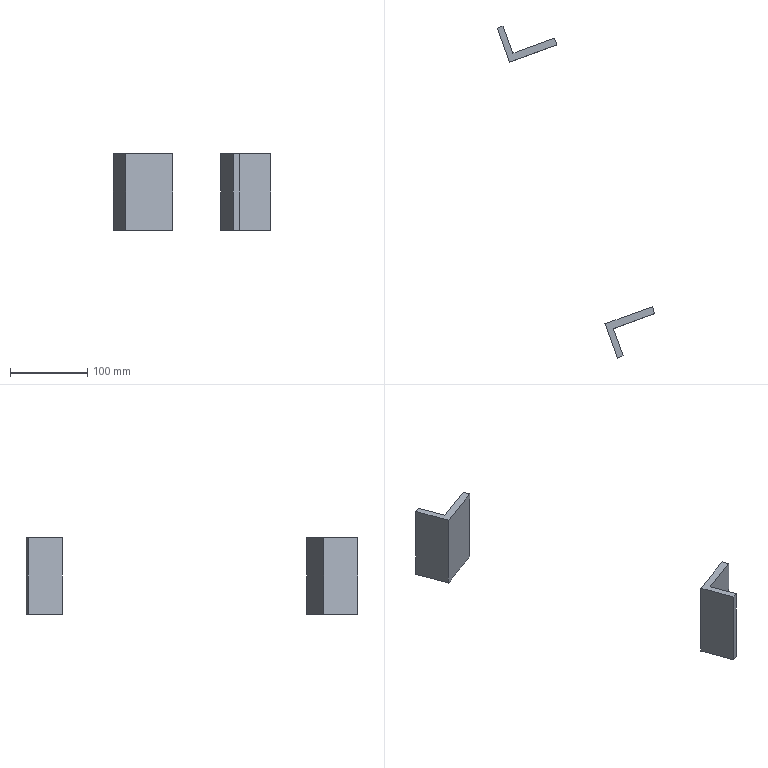Component | NX | MOUNTING_PLATE_2 | 2 solids | 16 faces | box 203.45 x 428.95 x 99.41 mm | volume 181780 mm3 | plane 16
STEP:
#1=CARTESIAN_POINT('',(0.,0.,0.));
#2=DIRECTION('',(0.,0.,1.));
#3=DIRECTION('',(1.,0.,0.));
#4=AXIS2_PLACEMENT_3D('',#1,#2,#3);
#5=CARTESIAN_POINT('',(-308.333,-604.49,-54.935));
#6=VERTEX_POINT('',#5);
#7=CARTESIAN_POINT('',(-308.333,-604.49,44.473));
#8=VERTEX_POINT('',#7);
#9=CARTESIAN_POINT('',(-308.333,-604.49,44.473));
#10=DIRECTION('',(0.,0.,1.));
#11=VECTOR('',#10,1.);
#12=LINE('',#9,#11);
#13=CARTESIAN_POINT('',(-298.936,-601.07,44.473));
#14=DIRECTION('',(0.342,-0.9397,0.));
#15=DIRECTION('',(0.,0.,1.));
#16=AXIS2_PLACEMENT_3D('',#13,#14,#15);
#17=PLANE('',#16);
#18=CARTESIAN_POINT('',(0.,10.));
#19=DIRECTION('',(1.,0.));
#20=VECTOR('',#19,1.);
#21=LINE('',#18,#20);
#22=(GEOMETRIC_REPRESENTATION_CONTEXT(2)PARAMETRIC_REPRESENTATION_CONTEXT()REPRESENTATION_CONTEXT('',''));
#23=DEFINITIONAL_REPRESENTATION('',(#21),#22);
#24=PCURVE('',#17,#23);
#25=CARTESIAN_POINT('',(56.842,-1607.798,0.));
#26=DIRECTION('',(0.9397,0.342,0.));
#27=DIRECTION('',(0.,0.,-1.));
#28=AXIS2_PLACEMENT_3D('',#25,#26,#27);
#29=PLANE('',#28);
#30=CARTESIAN_POINT('',(-44.473,1067.698));
#31=DIRECTION('',(-1.,0.));
#32=VECTOR('',#31,1.);
#33=LINE('',#30,#32);
#34=(GEOMETRIC_REPRESENTATION_CONTEXT(2)PARAMETRIC_REPRESENTATION_CONTEXT()REPRESENTATION_CONTEXT('',''));
#35=DEFINITIONAL_REPRESENTATION('',(#33),#34);
#36=PCURVE('',#29,#35);
#37=SURFACE_CURVE('',#12,(#24,#36),.PCURVE_S1.);
#38=EDGE_CURVE('',#6,#8,#37,.T.);
#39=ORIENTED_EDGE('',*,*,#38,.T.);
#40=CARTESIAN_POINT('',(-300.815,-601.754,44.473));
#41=VERTEX_POINT('',#40);
#42=CARTESIAN_POINT('',(-298.936,-601.07,44.473));
#43=DIRECTION('',(0.9397,0.342,0.));
#44=VECTOR('',#43,1.);
#45=LINE('',#42,#44);
#46=CARTESIAN_POINT('',(0.,0.));
#47=DIRECTION('',(0.,-1.));
#48=VECTOR('',#47,1.);
#49=LINE('',#46,#48);
#50=(GEOMETRIC_REPRESENTATION_CONTEXT(2)PARAMETRIC_REPRESENTATION_CONTEXT()REPRESENTATION_CONTEXT('',''));
#51=DEFINITIONAL_REPRESENTATION('',(#49),#50);
#52=PCURVE('',#17,#51);
#53=CARTESIAN_POINT('',(-287.544,-632.37,44.473));
#54=DIRECTION('',(0.,0.,-1.));
#55=DIRECTION('',(-0.9397,-0.342,0.));
#56=AXIS2_PLACEMENT_3D('',#53,#54,#55);
#57=PLANE('',#56);
#58=CARTESIAN_POINT('',(0.,33.308));
#59=DIRECTION('',(-1.,0.));
#60=VECTOR('',#59,1.);
#61=LINE('',#58,#60);
#62=(GEOMETRIC_REPRESENTATION_CONTEXT(2)PARAMETRIC_REPRESENTATION_CONTEXT()REPRESENTATION_CONTEXT('',''));
#63=DEFINITIONAL_REPRESENTATION('',(#61),#62);
#64=PCURVE('',#57,#63);
#65=SURFACE_CURVE('',#45,(#52,#64),.PCURVE_S1.);
#66=EDGE_CURVE('',#8,#41,#65,.T.);
#67=ORIENTED_EDGE('',*,*,#66,.T.);
#68=CARTESIAN_POINT('',(-300.815,-601.754,-54.935));
#69=VERTEX_POINT('',#68);
#70=CARTESIAN_POINT('',(-300.815,-601.754,44.473));
#71=DIRECTION('',(0.,0.,1.));
#72=VECTOR('',#71,1.);
#73=LINE('',#70,#72);
#74=CARTESIAN_POINT('',(0.,2.));
#75=DIRECTION('',(1.,0.));
#76=VECTOR('',#75,1.);
#77=LINE('',#74,#76);
#78=(GEOMETRIC_REPRESENTATION_CONTEXT(2)PARAMETRIC_REPRESENTATION_CONTEXT()REPRESENTATION_CONTEXT('',''));
#79=DEFINITIONAL_REPRESENTATION('',(#77),#78);
#80=PCURVE('',#17,#79);
#81=CARTESIAN_POINT('',(64.359,-1605.062,0.));
#82=DIRECTION('',(0.9397,0.342,0.));
#83=DIRECTION('',(0.,0.,-1.));
#84=AXIS2_PLACEMENT_3D('',#81,#82,#83);
#85=PLANE('',#84);
#86=CARTESIAN_POINT('',(-44.473,1067.698));
#87=DIRECTION('',(-1.,0.));
#88=VECTOR('',#87,1.);
#89=LINE('',#86,#88);
#90=(GEOMETRIC_REPRESENTATION_CONTEXT(2)PARAMETRIC_REPRESENTATION_CONTEXT()REPRESENTATION_CONTEXT('',''));
#91=DEFINITIONAL_REPRESENTATION('',(#89),#90);
#92=PCURVE('',#85,#91);
#93=SURFACE_CURVE('',#73,(#80,#92),.PCURVE_S1.);
#94=EDGE_CURVE('',#69,#41,#93,.T.);
#95=ORIENTED_EDGE('',*,*,#94,.F.);
#96=CARTESIAN_POINT('',(-298.936,-601.07,-54.935));
#97=DIRECTION('',(0.9397,0.342,0.));
#98=VECTOR('',#97,1.);
#99=LINE('',#96,#98);
#100=CARTESIAN_POINT('',(-99.408,0.));
#101=DIRECTION('',(0.,-1.));
#102=VECTOR('',#101,1.);
#103=LINE('',#100,#102);
#104=(GEOMETRIC_REPRESENTATION_CONTEXT(2)PARAMETRIC_REPRESENTATION_CONTEXT()REPRESENTATION_CONTEXT('',''));
#105=DEFINITIONAL_REPRESENTATION('',(#103),#104);
#106=PCURVE('',#17,#105);
#107=CARTESIAN_POINT('',(-298.936,-601.07,-54.935));
#108=DIRECTION('',(0.,0.,1.));
#109=DIRECTION('',(0.9397,0.342,0.));
#110=AXIS2_PLACEMENT_3D('',#107,#108,#109);
#111=PLANE('',#110);
#112=CARTESIAN_POINT('',(0.,0.));
#113=DIRECTION('',(1.,0.));
#114=VECTOR('',#113,1.);
#115=LINE('',#112,#114);
#116=(GEOMETRIC_REPRESENTATION_CONTEXT(2)PARAMETRIC_REPRESENTATION_CONTEXT()REPRESENTATION_CONTEXT('',''));
#117=DEFINITIONAL_REPRESENTATION('',(#115),#116);
#118=PCURVE('',#111,#117);
#119=SURFACE_CURVE('',#99,(#106,#118),.PCURVE_S1.);
#120=EDGE_CURVE('',#6,#69,#119,.T.);
#121=ORIENTED_EDGE('',*,*,#120,.F.);
#122=EDGE_LOOP('',(#39,#67,#95,#121));
#123=FACE_BOUND('',#122,.T.);
#124=ADVANCED_FACE('',(#123),#17,.F.);
#125=CARTESIAN_POINT('',(-292.332,-648.452,-54.935));
#126=VERTEX_POINT('',#125);
#127=CARTESIAN_POINT('',(-308.333,-604.49,-54.935));
#128=DIRECTION('',(-0.342,0.9397,0.));
#129=VECTOR('',#128,1.);
#130=LINE('',#127,#129);
#131=CARTESIAN_POINT('',(-10.,0.));
#132=DIRECTION('',(0.,1.));
#133=VECTOR('',#132,1.);
#134=LINE('',#131,#133);
#135=(GEOMETRIC_REPRESENTATION_CONTEXT(2)PARAMETRIC_REPRESENTATION_CONTEXT()REPRESENTATION_CONTEXT('',''));
#136=DEFINITIONAL_REPRESENTATION('',(#134),#135);
#137=PCURVE('',#111,#136);
#138=CARTESIAN_POINT('',(54.935,1067.698));
#139=DIRECTION('',(0.,1.));
#140=VECTOR('',#139,1.);
#141=LINE('',#138,#140);
#142=(GEOMETRIC_REPRESENTATION_CONTEXT(2)PARAMETRIC_REPRESENTATION_CONTEXT()REPRESENTATION_CONTEXT('',''));
#143=DEFINITIONAL_REPRESENTATION('',(#141),#142);
#144=PCURVE('',#29,#143);
#145=SURFACE_CURVE('',#130,(#137,#144),.PCURVE_S1.);
#146=EDGE_CURVE('',#126,#6,#145,.T.);
#147=ORIENTED_EDGE('',*,*,#146,.T.);
#148=ORIENTED_EDGE('',*,*,#120,.T.);
#149=CARTESIAN_POINT('',(-288.055,-636.813,-54.935));
#150=VERTEX_POINT('',#149);
#151=CARTESIAN_POINT('',(-300.815,-601.754,-54.935));
#152=DIRECTION('',(-0.342,0.9397,0.));
#153=VECTOR('',#152,1.);
#154=LINE('',#151,#153);
#155=CARTESIAN_POINT('',(-2.,0.));
#156=DIRECTION('',(0.,1.));
#157=VECTOR('',#156,1.);
#158=LINE('',#155,#157);
#159=(GEOMETRIC_REPRESENTATION_CONTEXT(2)PARAMETRIC_REPRESENTATION_CONTEXT()REPRESENTATION_CONTEXT('',''));
#160=DEFINITIONAL_REPRESENTATION('',(#158),#159);
#161=PCURVE('',#111,#160);
#162=CARTESIAN_POINT('',(54.935,1067.698));
#163=DIRECTION('',(0.,1.));
#164=VECTOR('',#163,1.);
#165=LINE('',#162,#164);
#166=(GEOMETRIC_REPRESENTATION_CONTEXT(2)PARAMETRIC_REPRESENTATION_CONTEXT()REPRESENTATION_CONTEXT('',''));
#167=DEFINITIONAL_REPRESENTATION('',(#165),#166);
#168=PCURVE('',#85,#167);
#169=SURFACE_CURVE('',#154,(#161,#168),.PCURVE_S1.);
#170=EDGE_CURVE('',#150,#69,#169,.T.);
#171=ORIENTED_EDGE('',*,*,#170,.F.);
#172=CARTESIAN_POINT('',(-234.492,-617.317,-54.935));
#173=VERTEX_POINT('',#172);
#174=CARTESIAN_POINT('',(-234.492,-617.317,-54.935));
#175=DIRECTION('',(0.9397,0.342,0.));
#176=VECTOR('',#175,1.);
#177=LINE('',#174,#176);
#178=CARTESIAN_POINT('',(55.,-37.308));
#179=DIRECTION('',(1.,0.));
#180=VECTOR('',#179,1.);
#181=LINE('',#178,#180);
#182=(GEOMETRIC_REPRESENTATION_CONTEXT(2)PARAMETRIC_REPRESENTATION_CONTEXT()REPRESENTATION_CONTEXT('',''));
#183=DEFINITIONAL_REPRESENTATION('',(#181),#182);
#184=PCURVE('',#111,#183);
#185=CARTESIAN_POINT('',(-234.492,-617.317,44.473));
#186=DIRECTION('',(0.342,-0.9397,0.));
#187=DIRECTION('',(0.,0.,1.));
#188=AXIS2_PLACEMENT_3D('',#185,#186,#187);
#189=PLANE('',#188);
#190=CARTESIAN_POINT('',(-99.408,0.));
#191=DIRECTION('',(0.,-1.));
#192=VECTOR('',#191,1.);
#193=LINE('',#190,#192);
#194=(GEOMETRIC_REPRESENTATION_CONTEXT(2)PARAMETRIC_REPRESENTATION_CONTEXT()REPRESENTATION_CONTEXT('',''));
#195=DEFINITIONAL_REPRESENTATION('',(#193),#194);
#196=PCURVE('',#189,#195);
#197=SURFACE_CURVE('',#177,(#184,#196),.PCURVE_S1.);
#198=EDGE_CURVE('',#150,#173,#197,.T.);
#199=ORIENTED_EDGE('',*,*,#198,.T.);
#200=CARTESIAN_POINT('',(-231.252,-626.221,-54.935));
#201=VERTEX_POINT('',#200);
#202=CARTESIAN_POINT('',(-235.86,-613.559,-54.935));
#203=DIRECTION('',(-0.342,0.9397,0.));
#204=VECTOR('',#203,1.);
#205=LINE('',#202,#204);
#206=CARTESIAN_POINT('',(55.,-33.308));
#207=DIRECTION('',(0.,1.));
#208=VECTOR('',#207,1.);
#209=LINE('',#206,#208);
#210=(GEOMETRIC_REPRESENTATION_CONTEXT(2)PARAMETRIC_REPRESENTATION_CONTEXT()REPRESENTATION_CONTEXT('',''));
#211=DEFINITIONAL_REPRESENTATION('',(#209),#210);
#212=PCURVE('',#111,#211);
#213=CARTESIAN_POINT('',(117.922,-1585.567,0.));
#214=DIRECTION('',(0.9397,0.342,0.));
#215=DIRECTION('',(0.,0.,-1.));
#216=AXIS2_PLACEMENT_3D('',#213,#214,#215);
#217=PLANE('',#216);
#218=CARTESIAN_POINT('',(54.935,1034.39));
#219=DIRECTION('',(0.,1.));
#220=VECTOR('',#219,1.);
#221=LINE('',#218,#220);
#222=(GEOMETRIC_REPRESENTATION_CONTEXT(2)PARAMETRIC_REPRESENTATION_CONTEXT()REPRESENTATION_CONTEXT('',''));
#223=DEFINITIONAL_REPRESENTATION('',(#221),#222);
#224=PCURVE('',#217,#223);
#225=SURFACE_CURVE('',#205,(#212,#224),.PCURVE_S1.);
#226=EDGE_CURVE('',#201,#173,#225,.T.);
#227=ORIENTED_EDGE('',*,*,#226,.F.);
#228=CARTESIAN_POINT('',(-231.252,-626.221,-54.935));
#229=DIRECTION('',(0.9397,0.342,0.));
#230=VECTOR('',#229,1.);
#231=LINE('',#228,#230);
#232=CARTESIAN_POINT('',(55.,-46.783));
#233=DIRECTION('',(1.,0.));
#234=VECTOR('',#233,1.);
#235=LINE('',#232,#234);
#236=(GEOMETRIC_REPRESENTATION_CONTEXT(2)PARAMETRIC_REPRESENTATION_CONTEXT()REPRESENTATION_CONTEXT('',''));
#237=DEFINITIONAL_REPRESENTATION('',(#235),#236);
#238=PCURVE('',#111,#237);
#239=CARTESIAN_POINT('',(-231.252,-626.221,-54.935));
#240=DIRECTION('',(-0.342,0.9397,0.));
#241=DIRECTION('',(0.,0.,-1.));
#242=AXIS2_PLACEMENT_3D('',#239,#240,#241);
#243=PLANE('',#242);
#244=CARTESIAN_POINT('',(0.,0.));
#245=DIRECTION('',(0.,-1.));
#246=VECTOR('',#245,1.);
#247=LINE('',#244,#246);
#248=(GEOMETRIC_REPRESENTATION_CONTEXT(2)PARAMETRIC_REPRESENTATION_CONTEXT()REPRESENTATION_CONTEXT('',''));
#249=DEFINITIONAL_REPRESENTATION('',(#247),#248);
#250=PCURVE('',#243,#249);
#251=SURFACE_CURVE('',#231,(#238,#250),.PCURVE_S1.);
#252=EDGE_CURVE('',#126,#201,#251,.T.);
#253=ORIENTED_EDGE('',*,*,#252,.F.);
#254=EDGE_LOOP('',(#147,#148,#171,#199,#227,#253));
#255=FACE_BOUND('',#254,.T.);
#256=ADVANCED_FACE('',(#255),#111,.F.);
#257=CARTESIAN_POINT('',(-292.332,-648.452,44.473));
#258=VERTEX_POINT('',#257);
#259=CARTESIAN_POINT('',(-296.94,-635.79,44.473));
#260=DIRECTION('',(0.342,-0.9397,0.));
#261=VECTOR('',#260,1.);
#262=LINE('',#259,#261);
#263=CARTESIAN_POINT('',(10.,0.));
#264=DIRECTION('',(0.,-1.));
#265=VECTOR('',#264,1.);
#266=LINE('',#263,#265);
#267=(GEOMETRIC_REPRESENTATION_CONTEXT(2)PARAMETRIC_REPRESENTATION_CONTEXT()REPRESENTATION_CONTEXT('',''));
#268=DEFINITIONAL_REPRESENTATION('',(#266),#267);
#269=PCURVE('',#57,#268);
#270=CARTESIAN_POINT('',(-44.473,1034.39));
#271=DIRECTION('',(0.,-1.));
#272=VECTOR('',#271,1.);
#273=LINE('',#270,#272);
#274=(GEOMETRIC_REPRESENTATION_CONTEXT(2)PARAMETRIC_REPRESENTATION_CONTEXT()REPRESENTATION_CONTEXT('',''));
#275=DEFINITIONAL_REPRESENTATION('',(#273),#274);
#276=PCURVE('',#29,#275);
#277=SURFACE_CURVE('',#262,(#269,#276),.PCURVE_S1.);
#278=EDGE_CURVE('',#8,#258,#277,.T.);
#279=ORIENTED_EDGE('',*,*,#278,.T.);
#280=CARTESIAN_POINT('',(-231.252,-626.221,44.473));
#281=VERTEX_POINT('',#280);
#282=CARTESIAN_POINT('',(-231.252,-626.221,44.473));
#283=DIRECTION('',(0.9397,0.342,0.));
#284=VECTOR('',#283,1.);
#285=LINE('',#282,#284);
#286=CARTESIAN_POINT('',(-55.,-13.475));
#287=DIRECTION('',(-1.,0.));
#288=VECTOR('',#287,1.);
#289=LINE('',#286,#288);
#290=(GEOMETRIC_REPRESENTATION_CONTEXT(2)PARAMETRIC_REPRESENTATION_CONTEXT()REPRESENTATION_CONTEXT('',''));
#291=DEFINITIONAL_REPRESENTATION('',(#289),#290);
#292=PCURVE('',#57,#291);
#293=CARTESIAN_POINT('',(-99.408,0.));
#294=DIRECTION('',(0.,-1.));
#295=VECTOR('',#294,1.);
#296=LINE('',#293,#295);
#297=(GEOMETRIC_REPRESENTATION_CONTEXT(2)PARAMETRIC_REPRESENTATION_CONTEXT()REPRESENTATION_CONTEXT('',''));
#298=DEFINITIONAL_REPRESENTATION('',(#296),#297);
#299=PCURVE('',#243,#298);
#300=SURFACE_CURVE('',#285,(#292,#299),.PCURVE_S1.);
#301=EDGE_CURVE('',#258,#281,#300,.T.);
#302=ORIENTED_EDGE('',*,*,#301,.T.);
#303=CARTESIAN_POINT('',(-234.492,-617.317,44.473));
#304=VERTEX_POINT('',#303);
#305=CARTESIAN_POINT('',(-231.252,-626.221,44.473));
#306=DIRECTION('',(0.342,-0.9397,0.));
#307=VECTOR('',#306,1.);
#308=LINE('',#305,#307);
#309=CARTESIAN_POINT('',(-55.,-13.475));
#310=DIRECTION('',(0.,-1.));
#311=VECTOR('',#310,1.);
#312=LINE('',#309,#311);
#313=(GEOMETRIC_REPRESENTATION_CONTEXT(2)PARAMETRIC_REPRESENTATION_CONTEXT()REPRESENTATION_CONTEXT('',''));
#314=DEFINITIONAL_REPRESENTATION('',(#312),#313);
#315=PCURVE('',#57,#314);
#316=CARTESIAN_POINT('',(-44.473,1020.915));
#317=DIRECTION('',(0.,-1.));
#318=VECTOR('',#317,1.);
#319=LINE('',#316,#318);
#320=(GEOMETRIC_REPRESENTATION_CONTEXT(2)PARAMETRIC_REPRESENTATION_CONTEXT()REPRESENTATION_CONTEXT('',''));
#321=DEFINITIONAL_REPRESENTATION('',(#319),#320);
#322=PCURVE('',#217,#321);
#323=SURFACE_CURVE('',#308,(#315,#322),.PCURVE_S1.);
#324=EDGE_CURVE('',#304,#281,#323,.T.);
#325=ORIENTED_EDGE('',*,*,#324,.F.);
#326=CARTESIAN_POINT('',(-288.055,-636.813,44.473));
#327=VERTEX_POINT('',#326);
#328=CARTESIAN_POINT('',(-234.492,-617.317,44.473));
#329=DIRECTION('',(0.9397,0.342,0.));
#330=VECTOR('',#329,1.);
#331=LINE('',#328,#330);
#332=CARTESIAN_POINT('',(-55.,-4.));
#333=DIRECTION('',(-1.,0.));
#334=VECTOR('',#333,1.);
#335=LINE('',#332,#334);
#336=(GEOMETRIC_REPRESENTATION_CONTEXT(2)PARAMETRIC_REPRESENTATION_CONTEXT()REPRESENTATION_CONTEXT('',''));
#337=DEFINITIONAL_REPRESENTATION('',(#335),#336);
#338=PCURVE('',#57,#337);
#339=CARTESIAN_POINT('',(0.,0.));
#340=DIRECTION('',(0.,-1.));
#341=VECTOR('',#340,1.);
#342=LINE('',#339,#341);
#343=(GEOMETRIC_REPRESENTATION_CONTEXT(2)PARAMETRIC_REPRESENTATION_CONTEXT()REPRESENTATION_CONTEXT('',''));
#344=DEFINITIONAL_REPRESENTATION('',(#342),#343);
#345=PCURVE('',#189,#344);
#346=SURFACE_CURVE('',#331,(#338,#345),.PCURVE_S1.);
#347=EDGE_CURVE('',#327,#304,#346,.T.);
#348=ORIENTED_EDGE('',*,*,#347,.F.);
#349=CARTESIAN_POINT('',(-289.423,-633.054,44.473));
#350=DIRECTION('',(0.342,-0.9397,0.));
#351=VECTOR('',#350,1.);
#352=LINE('',#349,#351);
#353=CARTESIAN_POINT('',(2.,0.));
#354=DIRECTION('',(0.,-1.));
#355=VECTOR('',#354,1.);
#356=LINE('',#353,#355);
#357=(GEOMETRIC_REPRESENTATION_CONTEXT(2)PARAMETRIC_REPRESENTATION_CONTEXT()REPRESENTATION_CONTEXT('',''));
#358=DEFINITIONAL_REPRESENTATION('',(#356),#357);
#359=PCURVE('',#57,#358);
#360=CARTESIAN_POINT('',(-44.473,1034.39));
#361=DIRECTION('',(0.,-1.));
#362=VECTOR('',#361,1.);
#363=LINE('',#360,#362);
#364=(GEOMETRIC_REPRESENTATION_CONTEXT(2)PARAMETRIC_REPRESENTATION_CONTEXT()REPRESENTATION_CONTEXT('',''));
#365=DEFINITIONAL_REPRESENTATION('',(#363),#364);
#366=PCURVE('',#85,#365);
#367=SURFACE_CURVE('',#352,(#359,#366),.PCURVE_S1.);
#368=EDGE_CURVE('',#41,#327,#367,.T.);
#369=ORIENTED_EDGE('',*,*,#368,.F.);
#370=ORIENTED_EDGE('',*,*,#66,.F.);
#371=EDGE_LOOP('',(#279,#302,#325,#348,#369,#370));
#372=FACE_BOUND('',#371,.T.);
#373=ADVANCED_FACE('',(#372),#57,.F.);
#374=ORIENTED_EDGE('',*,*,#94,.T.);
#375=ORIENTED_EDGE('',*,*,#368,.T.);
#376=CARTESIAN_POINT('',(-288.055,-636.813,-54.935));
#377=DIRECTION('',(0.,0.,-1.));
#378=VECTOR('',#377,1.);
#379=LINE('',#376,#378);
#380=CARTESIAN_POINT('',(54.935,1030.39));
#381=DIRECTION('',(1.,0.));
#382=VECTOR('',#381,1.);
#383=LINE('',#380,#382);
#384=(GEOMETRIC_REPRESENTATION_CONTEXT(2)PARAMETRIC_REPRESENTATION_CONTEXT()REPRESENTATION_CONTEXT('',''));
#385=DEFINITIONAL_REPRESENTATION('',(#383),#384);
#386=PCURVE('',#85,#385);
#387=CARTESIAN_POINT('',(-99.408,57.));
#388=DIRECTION('',(-1.,0.));
#389=VECTOR('',#388,1.);
#390=LINE('',#387,#389);
#391=(GEOMETRIC_REPRESENTATION_CONTEXT(2)PARAMETRIC_REPRESENTATION_CONTEXT()REPRESENTATION_CONTEXT('',''));
#392=DEFINITIONAL_REPRESENTATION('',(#390),#391);
#393=PCURVE('',#189,#392);
#394=SURFACE_CURVE('',#379,(#386,#393),.PCURVE_S1.);
#395=EDGE_CURVE('',#327,#150,#394,.T.);
#396=ORIENTED_EDGE('',*,*,#395,.T.);
#397=ORIENTED_EDGE('',*,*,#170,.T.);
#398=EDGE_LOOP('',(#374,#375,#396,#397));
#399=FACE_BOUND('',#398,.T.);
#400=ADVANCED_FACE('',(#399),#85,.T.);
#401=ORIENTED_EDGE('',*,*,#38,.F.);
#402=ORIENTED_EDGE('',*,*,#146,.F.);
#403=CARTESIAN_POINT('',(-292.332,-648.452,-54.935));
#404=DIRECTION('',(0.,0.,-1.));
#405=VECTOR('',#404,1.);
#406=LINE('',#403,#405);
#407=CARTESIAN_POINT('',(54.935,1020.915));
#408=DIRECTION('',(1.,0.));
#409=VECTOR('',#408,1.);
#410=LINE('',#407,#409);
#411=(GEOMETRIC_REPRESENTATION_CONTEXT(2)PARAMETRIC_REPRESENTATION_CONTEXT()REPRESENTATION_CONTEXT('',''));
#412=DEFINITIONAL_REPRESENTATION('',(#410),#411);
#413=PCURVE('',#29,#412);
#414=CARTESIAN_POINT('',(0.,65.));
#415=DIRECTION('',(1.,0.));
#416=VECTOR('',#415,1.);
#417=LINE('',#414,#416);
#418=(GEOMETRIC_REPRESENTATION_CONTEXT(2)PARAMETRIC_REPRESENTATION_CONTEXT()REPRESENTATION_CONTEXT('',''));
#419=DEFINITIONAL_REPRESENTATION('',(#417),#418);
#420=PCURVE('',#243,#419);
#421=SURFACE_CURVE('',#406,(#413,#420),.PCURVE_S1.);
#422=EDGE_CURVE('',#258,#126,#421,.T.);
#423=ORIENTED_EDGE('',*,*,#422,.F.);
#424=ORIENTED_EDGE('',*,*,#278,.F.);
#425=EDGE_LOOP('',(#401,#402,#423,#424));
#426=FACE_BOUND('',#425,.T.);
#427=ADVANCED_FACE('',(#426),#29,.F.);
#428=ORIENTED_EDGE('',*,*,#395,.F.);
#429=ORIENTED_EDGE('',*,*,#347,.T.);
#430=CARTESIAN_POINT('',(-234.492,-617.317,44.473));
#431=DIRECTION('',(0.,0.,1.));
#432=VECTOR('',#431,1.);
#433=LINE('',#430,#432);
#434=CARTESIAN_POINT('',(0.,0.));
#435=DIRECTION('',(1.,0.));
#436=VECTOR('',#435,1.);
#437=LINE('',#434,#436);
#438=(GEOMETRIC_REPRESENTATION_CONTEXT(2)PARAMETRIC_REPRESENTATION_CONTEXT()REPRESENTATION_CONTEXT('',''));
#439=DEFINITIONAL_REPRESENTATION('',(#437),#438);
#440=PCURVE('',#189,#439);
#441=CARTESIAN_POINT('',(-44.473,1030.39));
#442=DIRECTION('',(-1.,0.));
#443=VECTOR('',#442,1.);
#444=LINE('',#441,#443);
#445=(GEOMETRIC_REPRESENTATION_CONTEXT(2)PARAMETRIC_REPRESENTATION_CONTEXT()REPRESENTATION_CONTEXT('',''));
#446=DEFINITIONAL_REPRESENTATION('',(#444),#445);
#447=PCURVE('',#217,#446);
#448=SURFACE_CURVE('',#433,(#440,#447),.PCURVE_S1.);
#449=EDGE_CURVE('',#173,#304,#448,.T.);
#450=ORIENTED_EDGE('',*,*,#449,.F.);
#451=ORIENTED_EDGE('',*,*,#198,.F.);
#452=EDGE_LOOP('',(#428,#429,#450,#451));
#453=FACE_BOUND('',#452,.T.);
#454=ADVANCED_FACE('',(#453),#189,.F.);
#455=ORIENTED_EDGE('',*,*,#422,.T.);
#456=ORIENTED_EDGE('',*,*,#252,.T.);
#457=CARTESIAN_POINT('',(-231.252,-626.221,-54.935));
#458=DIRECTION('',(0.,0.,-1.));
#459=VECTOR('',#458,1.);
#460=LINE('',#457,#459);
#461=CARTESIAN_POINT('',(0.,0.));
#462=DIRECTION('',(1.,0.));
#463=VECTOR('',#462,1.);
#464=LINE('',#461,#463);
#465=(GEOMETRIC_REPRESENTATION_CONTEXT(2)PARAMETRIC_REPRESENTATION_CONTEXT()REPRESENTATION_CONTEXT('',''));
#466=DEFINITIONAL_REPRESENTATION('',(#464),#465);
#467=PCURVE('',#243,#466);
#468=CARTESIAN_POINT('',(54.935,1020.915));
#469=DIRECTION('',(1.,0.));
#470=VECTOR('',#469,1.);
#471=LINE('',#468,#470);
#472=(GEOMETRIC_REPRESENTATION_CONTEXT(2)PARAMETRIC_REPRESENTATION_CONTEXT()REPRESENTATION_CONTEXT('',''));
#473=DEFINITIONAL_REPRESENTATION('',(#471),#472);
#474=PCURVE('',#217,#473);
#475=SURFACE_CURVE('',#460,(#467,#474),.PCURVE_S1.);
#476=EDGE_CURVE('',#281,#201,#475,.T.);
#477=ORIENTED_EDGE('',*,*,#476,.F.);
#478=ORIENTED_EDGE('',*,*,#301,.F.);
#479=EDGE_LOOP('',(#455,#456,#477,#478));
#480=FACE_BOUND('',#479,.T.);
#481=ADVANCED_FACE('',(#480),#243,.F.);
#482=ORIENTED_EDGE('',*,*,#449,.T.);
#483=ORIENTED_EDGE('',*,*,#324,.T.);
#484=ORIENTED_EDGE('',*,*,#476,.T.);
#485=ORIENTED_EDGE('',*,*,#226,.T.);
#486=EDGE_LOOP('',(#482,#483,#484,#485));
#487=FACE_BOUND('',#486,.T.);
#488=ADVANCED_FACE('',(#487),#217,.T.);
#489=CLOSED_SHELL('',(#124,#256,#373,#400,#427,#454,#481,#488));
#490=MANIFOLD_SOLID_BREP('',#489);
#491=(LENGTH_UNIT()NAMED_UNIT(*)SI_UNIT(.MILLI.,.METRE.));
#492=UNCERTAINTY_MEASURE_WITH_UNIT(LENGTH_MEASURE(0.0000001),#491,'','');
#493=(NAMED_UNIT(*)PLANE_ANGLE_UNIT()SI_UNIT($,.RADIAN.));
#494=(NAMED_UNIT(*)SI_UNIT($,.STERADIAN.)SOLID_ANGLE_UNIT());
#495=(GEOMETRIC_REPRESENTATION_CONTEXT(3)GLOBAL_UNCERTAINTY_ASSIGNED_CONTEXT((#492))GLOBAL_UNIT_ASSIGNED_CONTEXT((#491,#493,#494))REPRESENTATION_CONTEXT('',''));
#496=ADVANCED_BREP_SHAPE_REPRESENTATION('',(#4,#490),#495);
#497=CARTESIAN_POINT('',(0.,0.,0.));
#498=DIRECTION('',(0.,0.,1.));
#499=DIRECTION('',(1.,0.,0.));
#500=AXIS2_PLACEMENT_3D('',#497,#498,#499);
#501=CARTESIAN_POINT('',(0.,0.,0.));
#502=DIRECTION('',(0.,0.,1.));
#503=DIRECTION('',(1.,0.,0.));
#504=AXIS2_PLACEMENT_3D('',#501,#502,#503);
#505=(LENGTH_UNIT()NAMED_UNIT(*)SI_UNIT(.MILLI.,.METRE.));
#506=UNCERTAINTY_MEASURE_WITH_UNIT(LENGTH_MEASURE(0.0000001),#505,'','');
#507=(NAMED_UNIT(*)PLANE_ANGLE_UNIT()SI_UNIT($,.RADIAN.));
#508=(NAMED_UNIT(*)SI_UNIT($,.STERADIAN.)SOLID_ANGLE_UNIT());
#509=(GEOMETRIC_REPRESENTATION_CONTEXT(3)GLOBAL_UNCERTAINTY_ASSIGNED_CONTEXT((#506))GLOBAL_UNIT_ASSIGNED_CONTEXT((#505,#507,#508))REPRESENTATION_CONTEXT('',''));
#510=SHAPE_REPRESENTATION('',(#4,#500,#504),#509);
#511=ITEM_DEFINED_TRANSFORMATION('','',#4,#500);
#512=(REPRESENTATION_RELATIONSHIP('','',#496,#510)REPRESENTATION_RELATIONSHIP_WITH_TRANSFORMATION(#511)SHAPE_REPRESENTATION_RELATIONSHIP());
#513=CARTESIAN_POINT('',(-153.204,-1030.703,44.473));
#514=VERTEX_POINT('',#513);
#515=CARTESIAN_POINT('',(-153.204,-1030.703,-54.935));
#516=VERTEX_POINT('',#515);
#517=CARTESIAN_POINT('',(-153.204,-1030.703,44.473));
#518=DIRECTION('',(0.,0.,-1.));
#519=VECTOR('',#518,1.);
#520=LINE('',#517,#519);
#521=CARTESIAN_POINT('',(-143.807,-1027.283,44.473));
#522=DIRECTION('',(-0.342,0.9397,0.));
#523=DIRECTION('',(0.,0.,1.));
#524=AXIS2_PLACEMENT_3D('',#521,#522,#523);
#525=PLANE('',#524);
#526=CARTESIAN_POINT('',(0.,-10.));
#527=DIRECTION('',(-1.,0.));
#528=VECTOR('',#527,1.);
#529=LINE('',#526,#528);
#530=(GEOMETRIC_REPRESENTATION_CONTEXT(2)PARAMETRIC_REPRESENTATION_CONTEXT()REPRESENTATION_CONTEXT('',''));
#531=DEFINITIONAL_REPRESENTATION('',(#529),#530);
#532=PCURVE('',#525,#531);
#533=CARTESIAN_POINT('',(-518.378,-27.395,0.));
#534=DIRECTION('',(0.9397,0.342,0.));
#535=DIRECTION('',(0.,0.,-1.));
#536=AXIS2_PLACEMENT_3D('',#533,#534,#535);
#537=PLANE('',#536);
#538=CARTESIAN_POINT('',(-44.473,-1067.698));
#539=DIRECTION('',(1.,0.));
#540=VECTOR('',#539,1.);
#541=LINE('',#538,#540);
#542=(GEOMETRIC_REPRESENTATION_CONTEXT(2)PARAMETRIC_REPRESENTATION_CONTEXT()REPRESENTATION_CONTEXT('',''));
#543=DEFINITIONAL_REPRESENTATION('',(#541),#542);
#544=PCURVE('',#537,#543);
#545=SURFACE_CURVE('',#520,(#532,#544),.PCURVE_S1.);
#546=EDGE_CURVE('',#514,#516,#545,.T.);
#547=ORIENTED_EDGE('',*,*,#546,.T.);
#548=CARTESIAN_POINT('',(-145.686,-1027.967,-54.935));
#549=VERTEX_POINT('',#548);
#550=CARTESIAN_POINT('',(-143.807,-1027.283,-54.935));
#551=DIRECTION('',(-0.9397,-0.342,0.));
#552=VECTOR('',#551,1.);
#553=LINE('',#550,#552);
#554=CARTESIAN_POINT('',(-99.408,0.));
#555=DIRECTION('',(0.,-1.));
#556=VECTOR('',#555,1.);
#557=LINE('',#554,#556);
#558=(GEOMETRIC_REPRESENTATION_CONTEXT(2)PARAMETRIC_REPRESENTATION_CONTEXT()REPRESENTATION_CONTEXT('',''));
#559=DEFINITIONAL_REPRESENTATION('',(#557),#558);
#560=PCURVE('',#525,#559);
#561=CARTESIAN_POINT('',(-143.807,-1027.283,-54.935));
#562=DIRECTION('',(0.,0.,1.));
#563=DIRECTION('',(0.9397,0.342,0.));
#564=AXIS2_PLACEMENT_3D('',#561,#562,#563);
#565=PLANE('',#564);
#566=CARTESIAN_POINT('',(0.,0.));
#567=DIRECTION('',(-1.,0.));
#568=VECTOR('',#567,1.);
#569=LINE('',#566,#568);
#570=(GEOMETRIC_REPRESENTATION_CONTEXT(2)PARAMETRIC_REPRESENTATION_CONTEXT()REPRESENTATION_CONTEXT('',''));
#571=DEFINITIONAL_REPRESENTATION('',(#569),#570);
#572=PCURVE('',#565,#571);
#573=SURFACE_CURVE('',#553,(#560,#572),.PCURVE_S1.);
#574=EDGE_CURVE('',#549,#516,#573,.T.);
#575=ORIENTED_EDGE('',*,*,#574,.F.);
#576=CARTESIAN_POINT('',(-145.686,-1027.967,44.473));
#577=VERTEX_POINT('',#576);
#578=CARTESIAN_POINT('',(-145.686,-1027.967,44.473));
#579=DIRECTION('',(0.,0.,-1.));
#580=VECTOR('',#579,1.);
#581=LINE('',#578,#580);
#582=CARTESIAN_POINT('',(0.,-2.));
#583=DIRECTION('',(-1.,0.));
#584=VECTOR('',#583,1.);
#585=LINE('',#582,#584);
#586=(GEOMETRIC_REPRESENTATION_CONTEXT(2)PARAMETRIC_REPRESENTATION_CONTEXT()REPRESENTATION_CONTEXT('',''));
#587=DEFINITIONAL_REPRESENTATION('',(#585),#586);
#588=PCURVE('',#525,#587);
#589=CARTESIAN_POINT('',(-510.861,-24.659,0.));
#590=DIRECTION('',(0.9397,0.342,0.));
#591=DIRECTION('',(0.,0.,-1.));
#592=AXIS2_PLACEMENT_3D('',#589,#590,#591);
#593=PLANE('',#592);
#594=CARTESIAN_POINT('',(-44.473,-1067.698));
#595=DIRECTION('',(1.,0.));
#596=VECTOR('',#595,1.);
#597=LINE('',#594,#596);
#598=(GEOMETRIC_REPRESENTATION_CONTEXT(2)PARAMETRIC_REPRESENTATION_CONTEXT()REPRESENTATION_CONTEXT('',''));
#599=DEFINITIONAL_REPRESENTATION('',(#597),#598);
#600=PCURVE('',#593,#599);
#601=SURFACE_CURVE('',#581,(#588,#600),.PCURVE_S1.);
#602=EDGE_CURVE('',#577,#549,#601,.T.);
#603=ORIENTED_EDGE('',*,*,#602,.F.);
#604=CARTESIAN_POINT('',(-143.807,-1027.283,44.473));
#605=DIRECTION('',(-0.9397,-0.342,0.));
#606=VECTOR('',#605,1.);
#607=LINE('',#604,#606);
#608=CARTESIAN_POINT('',(0.,0.));
#609=DIRECTION('',(0.,-1.));
#610=VECTOR('',#609,1.);
#611=LINE('',#608,#610);
#612=(GEOMETRIC_REPRESENTATION_CONTEXT(2)PARAMETRIC_REPRESENTATION_CONTEXT()REPRESENTATION_CONTEXT('',''));
#613=DEFINITIONAL_REPRESENTATION('',(#611),#612);
#614=PCURVE('',#525,#613);
#615=CARTESIAN_POINT('',(-155.199,-995.983,44.473));
#616=DIRECTION('',(0.,0.,-1.));
#617=DIRECTION('',(-0.9397,-0.342,0.));
#618=AXIS2_PLACEMENT_3D('',#615,#616,#617);
#619=PLANE('',#618);
#620=CARTESIAN_POINT('',(-0.,-33.308));
#621=DIRECTION('',(1.,-0.));
#622=VECTOR('',#621,1.);
#623=LINE('',#620,#622);
#624=(GEOMETRIC_REPRESENTATION_CONTEXT(2)PARAMETRIC_REPRESENTATION_CONTEXT()REPRESENTATION_CONTEXT('',''));
#625=DEFINITIONAL_REPRESENTATION('',(#623),#624);
#626=PCURVE('',#619,#625);
#627=SURFACE_CURVE('',#607,(#614,#626),.PCURVE_S1.);
#628=EDGE_CURVE('',#577,#514,#627,.T.);
#629=ORIENTED_EDGE('',*,*,#628,.T.);
#630=EDGE_LOOP('',(#547,#575,#603,#629));
#631=FACE_BOUND('',#630,.T.);
#632=ADVANCED_FACE('',(#631),#525,.F.);
#633=CARTESIAN_POINT('',(-169.205,-986.741,-54.935));
#634=VERTEX_POINT('',#633);
#635=CARTESIAN_POINT('',(-153.204,-1030.703,-54.935));
#636=DIRECTION('',(-0.342,0.9397,0.));
#637=VECTOR('',#636,1.);
#638=LINE('',#635,#637);
#639=CARTESIAN_POINT('',(-10.,-0.));
#640=DIRECTION('',(0.,1.));
#641=VECTOR('',#640,1.);
#642=LINE('',#639,#641);
#643=(GEOMETRIC_REPRESENTATION_CONTEXT(2)PARAMETRIC_REPRESENTATION_CONTEXT()REPRESENTATION_CONTEXT('',''));
#644=DEFINITIONAL_REPRESENTATION('',(#642),#643);
#645=PCURVE('',#565,#644);
#646=CARTESIAN_POINT('',(54.935,-1067.698));
#647=DIRECTION('',(0.,1.));
#648=VECTOR('',#647,1.);
#649=LINE('',#646,#648);
#650=(GEOMETRIC_REPRESENTATION_CONTEXT(2)PARAMETRIC_REPRESENTATION_CONTEXT()REPRESENTATION_CONTEXT('',''));
#651=DEFINITIONAL_REPRESENTATION('',(#649),#650);
#652=PCURVE('',#537,#651);
#653=SURFACE_CURVE('',#638,(#645,#652),.PCURVE_S1.);
#654=EDGE_CURVE('',#516,#634,#653,.T.);
#655=ORIENTED_EDGE('',*,*,#654,.T.);
#656=CARTESIAN_POINT('',(-108.125,-964.51,-54.935));
#657=VERTEX_POINT('',#656);
#658=CARTESIAN_POINT('',(-108.125,-964.51,-54.935));
#659=DIRECTION('',(-0.9397,-0.342,0.));
#660=VECTOR('',#659,1.);
#661=LINE('',#658,#660);
#662=CARTESIAN_POINT('',(55.,46.783));
#663=DIRECTION('',(-1.,0.));
#664=VECTOR('',#663,1.);
#665=LINE('',#662,#664);
#666=(GEOMETRIC_REPRESENTATION_CONTEXT(2)PARAMETRIC_REPRESENTATION_CONTEXT()REPRESENTATION_CONTEXT('',''));
#667=DEFINITIONAL_REPRESENTATION('',(#665),#666);
#668=PCURVE('',#565,#667);
#669=CARTESIAN_POINT('',(-108.125,-964.51,-54.935));
#670=DIRECTION('',(0.342,-0.9397,0.));
#671=DIRECTION('',(0.,0.,-1.));
#672=AXIS2_PLACEMENT_3D('',#669,#670,#671);
#673=PLANE('',#672);
#674=CARTESIAN_POINT('',(0.,0.));
#675=DIRECTION('',(0.,-1.));
#676=VECTOR('',#675,1.);
#677=LINE('',#674,#676);
#678=(GEOMETRIC_REPRESENTATION_CONTEXT(2)PARAMETRIC_REPRESENTATION_CONTEXT()REPRESENTATION_CONTEXT('',''));
#679=DEFINITIONAL_REPRESENTATION('',(#677),#678);
#680=PCURVE('',#673,#679);
#681=SURFACE_CURVE('',#661,(#668,#680),.PCURVE_S1.);
#682=EDGE_CURVE('',#657,#634,#681,.T.);
#683=ORIENTED_EDGE('',*,*,#682,.F.);
#684=CARTESIAN_POINT('',(-104.884,-973.413,-54.935));
#685=VERTEX_POINT('',#684);
#686=CARTESIAN_POINT('',(-103.516,-977.172,-54.935));
#687=DIRECTION('',(-0.342,0.9397,0.));
#688=VECTOR('',#687,1.);
#689=LINE('',#686,#688);
#690=CARTESIAN_POINT('',(55.,33.308));
#691=DIRECTION('',(0.,1.));
#692=VECTOR('',#691,1.);
#693=LINE('',#690,#692);
#694=(GEOMETRIC_REPRESENTATION_CONTEXT(2)PARAMETRIC_REPRESENTATION_CONTEXT()REPRESENTATION_CONTEXT('',''));
#695=DEFINITIONAL_REPRESENTATION('',(#693),#694);
#696=PCURVE('',#565,#695);
#697=CARTESIAN_POINT('',(-457.298,-5.164,0.));
#698=DIRECTION('',(0.9397,0.342,0.));
#699=DIRECTION('',(0.,0.,-1.));
#700=AXIS2_PLACEMENT_3D('',#697,#698,#699);
#701=PLANE('',#700);
#702=CARTESIAN_POINT('',(54.935,-1034.39));
#703=DIRECTION('',(0.,1.));
#704=VECTOR('',#703,1.);
#705=LINE('',#702,#704);
#706=(GEOMETRIC_REPRESENTATION_CONTEXT(2)PARAMETRIC_REPRESENTATION_CONTEXT()REPRESENTATION_CONTEXT('',''));
#707=DEFINITIONAL_REPRESENTATION('',(#705),#706);
#708=PCURVE('',#701,#707);
#709=SURFACE_CURVE('',#689,(#696,#708),.PCURVE_S1.);
#710=EDGE_CURVE('',#685,#657,#709,.T.);
#711=ORIENTED_EDGE('',*,*,#710,.F.);
#712=CARTESIAN_POINT('',(-158.447,-992.908,-54.935));
#713=VERTEX_POINT('',#712);
#714=CARTESIAN_POINT('',(-104.884,-973.413,-54.935));
#715=DIRECTION('',(-0.9397,-0.342,0.));
#716=VECTOR('',#715,1.);
#717=LINE('',#714,#716);
#718=CARTESIAN_POINT('',(55.,37.308));
#719=DIRECTION('',(-1.,0.));
#720=VECTOR('',#719,1.);
#721=LINE('',#718,#720);
#722=(GEOMETRIC_REPRESENTATION_CONTEXT(2)PARAMETRIC_REPRESENTATION_CONTEXT()REPRESENTATION_CONTEXT('',''));
#723=DEFINITIONAL_REPRESENTATION('',(#721),#722);
#724=PCURVE('',#565,#723);
#725=CARTESIAN_POINT('',(-104.884,-973.413,44.473));
#726=DIRECTION('',(-0.342,0.9397,0.));
#727=DIRECTION('',(0.,0.,1.));
#728=AXIS2_PLACEMENT_3D('',#725,#726,#727);
#729=PLANE('',#728);
#730=CARTESIAN_POINT('',(-99.408,0.));
#731=DIRECTION('',(0.,-1.));
#732=VECTOR('',#731,1.);
#733=LINE('',#730,#732);
#734=(GEOMETRIC_REPRESENTATION_CONTEXT(2)PARAMETRIC_REPRESENTATION_CONTEXT()REPRESENTATION_CONTEXT('',''));
#735=DEFINITIONAL_REPRESENTATION('',(#733),#734);
#736=PCURVE('',#729,#735);
#737=SURFACE_CURVE('',#717,(#724,#736),.PCURVE_S1.);
#738=EDGE_CURVE('',#685,#713,#737,.T.);
#739=ORIENTED_EDGE('',*,*,#738,.T.);
#740=CARTESIAN_POINT('',(-145.686,-1027.967,-54.935));
#741=DIRECTION('',(-0.342,0.9397,0.));
#742=VECTOR('',#741,1.);
#743=LINE('',#740,#742);
#744=CARTESIAN_POINT('',(-2.,0.));
#745=DIRECTION('',(0.,1.));
#746=VECTOR('',#745,1.);
#747=LINE('',#744,#746);
#748=(GEOMETRIC_REPRESENTATION_CONTEXT(2)PARAMETRIC_REPRESENTATION_CONTEXT()REPRESENTATION_CONTEXT('',''));
#749=DEFINITIONAL_REPRESENTATION('',(#747),#748);
#750=PCURVE('',#565,#749);
#751=CARTESIAN_POINT('',(54.935,-1067.698));
#752=DIRECTION('',(0.,1.));
#753=VECTOR('',#752,1.);
#754=LINE('',#751,#753);
#755=(GEOMETRIC_REPRESENTATION_CONTEXT(2)PARAMETRIC_REPRESENTATION_CONTEXT()REPRESENTATION_CONTEXT('',''));
#756=DEFINITIONAL_REPRESENTATION('',(#754),#755);
#757=PCURVE('',#593,#756);
#758=SURFACE_CURVE('',#743,(#750,#757),.PCURVE_S1.);
#759=EDGE_CURVE('',#549,#713,#758,.T.);
#760=ORIENTED_EDGE('',*,*,#759,.F.);
#761=ORIENTED_EDGE('',*,*,#574,.T.);
#762=EDGE_LOOP('',(#655,#683,#711,#739,#760,#761));
#763=FACE_BOUND('',#762,.T.);
#764=ADVANCED_FACE('',(#763),#565,.F.);
#765=CARTESIAN_POINT('',(-169.205,-986.741,44.473));
#766=VERTEX_POINT('',#765);
#767=CARTESIAN_POINT('',(-164.596,-999.403,44.473));
#768=DIRECTION('',(0.342,-0.9397,0.));
#769=VECTOR('',#768,1.);
#770=LINE('',#767,#769);
#771=CARTESIAN_POINT('',(10.,0.));
#772=DIRECTION('',(-0.,-1.));
#773=VECTOR('',#772,1.);
#774=LINE('',#771,#773);
#775=(GEOMETRIC_REPRESENTATION_CONTEXT(2)PARAMETRIC_REPRESENTATION_CONTEXT()REPRESENTATION_CONTEXT('',''));
#776=DEFINITIONAL_REPRESENTATION('',(#774),#775);
#777=PCURVE('',#619,#776);
#778=CARTESIAN_POINT('',(-44.473,-1034.39));
#779=DIRECTION('',(0.,-1.));
#780=VECTOR('',#779,1.);
#781=LINE('',#778,#780);
#782=(GEOMETRIC_REPRESENTATION_CONTEXT(2)PARAMETRIC_REPRESENTATION_CONTEXT()REPRESENTATION_CONTEXT('',''));
#783=DEFINITIONAL_REPRESENTATION('',(#781),#782);
#784=PCURVE('',#537,#783);
#785=SURFACE_CURVE('',#770,(#777,#784),.PCURVE_S1.);
#786=EDGE_CURVE('',#766,#514,#785,.T.);
#787=ORIENTED_EDGE('',*,*,#786,.T.);
#788=ORIENTED_EDGE('',*,*,#628,.F.);
#789=CARTESIAN_POINT('',(-158.447,-992.908,44.473));
#790=VERTEX_POINT('',#789);
#791=CARTESIAN_POINT('',(-157.079,-996.667,44.473));
#792=DIRECTION('',(0.342,-0.9397,0.));
#793=VECTOR('',#792,1.);
#794=LINE('',#791,#793);
#795=CARTESIAN_POINT('',(2.,0.));
#796=DIRECTION('',(-0.,-1.));
#797=VECTOR('',#796,1.);
#798=LINE('',#795,#797);
#799=(GEOMETRIC_REPRESENTATION_CONTEXT(2)PARAMETRIC_REPRESENTATION_CONTEXT()REPRESENTATION_CONTEXT('',''));
#800=DEFINITIONAL_REPRESENTATION('',(#798),#799);
#801=PCURVE('',#619,#800);
#802=CARTESIAN_POINT('',(-44.473,-1034.39));
#803=DIRECTION('',(0.,-1.));
#804=VECTOR('',#803,1.);
#805=LINE('',#802,#804);
#806=(GEOMETRIC_REPRESENTATION_CONTEXT(2)PARAMETRIC_REPRESENTATION_CONTEXT()REPRESENTATION_CONTEXT('',''));
#807=DEFINITIONAL_REPRESENTATION('',(#805),#806);
#808=PCURVE('',#593,#807);
#809=SURFACE_CURVE('',#794,(#801,#808),.PCURVE_S1.);
#810=EDGE_CURVE('',#790,#577,#809,.T.);
#811=ORIENTED_EDGE('',*,*,#810,.F.);
#812=CARTESIAN_POINT('',(-104.884,-973.413,44.473));
#813=VERTEX_POINT('',#812);
#814=CARTESIAN_POINT('',(-104.884,-973.413,44.473));
#815=DIRECTION('',(-0.9397,-0.342,0.));
#816=VECTOR('',#815,1.);
#817=LINE('',#814,#816);
#818=CARTESIAN_POINT('',(-55.,4.));
#819=DIRECTION('',(1.,-0.));
#820=VECTOR('',#819,1.);
#821=LINE('',#818,#820);
#822=(GEOMETRIC_REPRESENTATION_CONTEXT(2)PARAMETRIC_REPRESENTATION_CONTEXT()REPRESENTATION_CONTEXT('',''));
#823=DEFINITIONAL_REPRESENTATION('',(#821),#822);
#824=PCURVE('',#619,#823);
#825=CARTESIAN_POINT('',(0.,0.));
#826=DIRECTION('',(0.,-1.));
#827=VECTOR('',#826,1.);
#828=LINE('',#825,#827);
#829=(GEOMETRIC_REPRESENTATION_CONTEXT(2)PARAMETRIC_REPRESENTATION_CONTEXT()REPRESENTATION_CONTEXT('',''));
#830=DEFINITIONAL_REPRESENTATION('',(#828),#829);
#831=PCURVE('',#729,#830);
#832=SURFACE_CURVE('',#817,(#824,#831),.PCURVE_S1.);
#833=EDGE_CURVE('',#813,#790,#832,.T.);
#834=ORIENTED_EDGE('',*,*,#833,.F.);
#835=CARTESIAN_POINT('',(-108.125,-964.51,44.473));
#836=VERTEX_POINT('',#835);
#837=CARTESIAN_POINT('',(-108.125,-964.51,44.473));
#838=DIRECTION('',(0.342,-0.9397,0.));
#839=VECTOR('',#838,1.);
#840=LINE('',#837,#839);
#841=CARTESIAN_POINT('',(-55.,13.475));
#842=DIRECTION('',(-0.,-1.));
#843=VECTOR('',#842,1.);
#844=LINE('',#841,#843);
#845=(GEOMETRIC_REPRESENTATION_CONTEXT(2)PARAMETRIC_REPRESENTATION_CONTEXT()REPRESENTATION_CONTEXT('',''));
#846=DEFINITIONAL_REPRESENTATION('',(#844),#845);
#847=PCURVE('',#619,#846);
#848=CARTESIAN_POINT('',(-44.473,-1020.915));
#849=DIRECTION('',(0.,-1.));
#850=VECTOR('',#849,1.);
#851=LINE('',#848,#850);
#852=(GEOMETRIC_REPRESENTATION_CONTEXT(2)PARAMETRIC_REPRESENTATION_CONTEXT()REPRESENTATION_CONTEXT('',''));
#853=DEFINITIONAL_REPRESENTATION('',(#851),#852);
#854=PCURVE('',#701,#853);
#855=SURFACE_CURVE('',#840,(#847,#854),.PCURVE_S1.);
#856=EDGE_CURVE('',#836,#813,#855,.T.);
#857=ORIENTED_EDGE('',*,*,#856,.F.);
#858=CARTESIAN_POINT('',(-108.125,-964.51,44.473));
#859=DIRECTION('',(-0.9397,-0.342,0.));
#860=VECTOR('',#859,1.);
#861=LINE('',#858,#860);
#862=CARTESIAN_POINT('',(-55.,13.475));
#863=DIRECTION('',(1.,-0.));
#864=VECTOR('',#863,1.);
#865=LINE('',#862,#864);
#866=(GEOMETRIC_REPRESENTATION_CONTEXT(2)PARAMETRIC_REPRESENTATION_CONTEXT()REPRESENTATION_CONTEXT('',''));
#867=DEFINITIONAL_REPRESENTATION('',(#865),#866);
#868=PCURVE('',#619,#867);
#869=CARTESIAN_POINT('',(-99.408,0.));
#870=DIRECTION('',(0.,-1.));
#871=VECTOR('',#870,1.);
#872=LINE('',#869,#871);
#873=(GEOMETRIC_REPRESENTATION_CONTEXT(2)PARAMETRIC_REPRESENTATION_CONTEXT()REPRESENTATION_CONTEXT('',''));
#874=DEFINITIONAL_REPRESENTATION('',(#872),#873);
#875=PCURVE('',#673,#874);
#876=SURFACE_CURVE('',#861,(#868,#875),.PCURVE_S1.);
#877=EDGE_CURVE('',#836,#766,#876,.T.);
#878=ORIENTED_EDGE('',*,*,#877,.T.);
#879=EDGE_LOOP('',(#787,#788,#811,#834,#857,#878));
#880=FACE_BOUND('',#879,.T.);
#881=ADVANCED_FACE('',(#880),#619,.F.);
#882=ORIENTED_EDGE('',*,*,#602,.T.);
#883=ORIENTED_EDGE('',*,*,#759,.T.);
#884=CARTESIAN_POINT('',(-158.447,-992.908,-54.935));
#885=DIRECTION('',(0.,0.,1.));
#886=VECTOR('',#885,1.);
#887=LINE('',#884,#886);
#888=CARTESIAN_POINT('',(54.935,-1030.39));
#889=DIRECTION('',(-1.,0.));
#890=VECTOR('',#889,1.);
#891=LINE('',#888,#890);
#892=(GEOMETRIC_REPRESENTATION_CONTEXT(2)PARAMETRIC_REPRESENTATION_CONTEXT()REPRESENTATION_CONTEXT('',''));
#893=DEFINITIONAL_REPRESENTATION('',(#891),#892);
#894=PCURVE('',#593,#893);
#895=CARTESIAN_POINT('',(-99.408,-57.));
#896=DIRECTION('',(1.,0.));
#897=VECTOR('',#896,1.);
#898=LINE('',#895,#897);
#899=(GEOMETRIC_REPRESENTATION_CONTEXT(2)PARAMETRIC_REPRESENTATION_CONTEXT()REPRESENTATION_CONTEXT('',''));
#900=DEFINITIONAL_REPRESENTATION('',(#898),#899);
#901=PCURVE('',#729,#900);
#902=SURFACE_CURVE('',#887,(#894,#901),.PCURVE_S1.);
#903=EDGE_CURVE('',#713,#790,#902,.T.);
#904=ORIENTED_EDGE('',*,*,#903,.T.);
#905=ORIENTED_EDGE('',*,*,#810,.T.);
#906=EDGE_LOOP('',(#882,#883,#904,#905));
#907=FACE_BOUND('',#906,.T.);
#908=ADVANCED_FACE('',(#907),#593,.T.);
#909=ORIENTED_EDGE('',*,*,#546,.F.);
#910=ORIENTED_EDGE('',*,*,#786,.F.);
#911=CARTESIAN_POINT('',(-169.205,-986.741,-54.935));
#912=DIRECTION('',(0.,0.,1.));
#913=VECTOR('',#912,1.);
#914=LINE('',#911,#913);
#915=CARTESIAN_POINT('',(54.935,-1020.915));
#916=DIRECTION('',(-1.,0.));
#917=VECTOR('',#916,1.);
#918=LINE('',#915,#917);
#919=(GEOMETRIC_REPRESENTATION_CONTEXT(2)PARAMETRIC_REPRESENTATION_CONTEXT()REPRESENTATION_CONTEXT('',''));
#920=DEFINITIONAL_REPRESENTATION('',(#918),#919);
#921=PCURVE('',#537,#920);
#922=CARTESIAN_POINT('',(0.,-65.));
#923=DIRECTION('',(-1.,0.));
#924=VECTOR('',#923,1.);
#925=LINE('',#922,#924);
#926=(GEOMETRIC_REPRESENTATION_CONTEXT(2)PARAMETRIC_REPRESENTATION_CONTEXT()REPRESENTATION_CONTEXT('',''));
#927=DEFINITIONAL_REPRESENTATION('',(#925),#926);
#928=PCURVE('',#673,#927);
#929=SURFACE_CURVE('',#914,(#921,#928),.PCURVE_S1.);
#930=EDGE_CURVE('',#634,#766,#929,.T.);
#931=ORIENTED_EDGE('',*,*,#930,.F.);
#932=ORIENTED_EDGE('',*,*,#654,.F.);
#933=EDGE_LOOP('',(#909,#910,#931,#932));
#934=FACE_BOUND('',#933,.T.);
#935=ADVANCED_FACE('',(#934),#537,.F.);
#936=ORIENTED_EDGE('',*,*,#903,.F.);
#937=ORIENTED_EDGE('',*,*,#738,.F.);
#938=CARTESIAN_POINT('',(-104.884,-973.413,44.473));
#939=DIRECTION('',(0.,0.,-1.));
#940=VECTOR('',#939,1.);
#941=LINE('',#938,#940);
#942=CARTESIAN_POINT('',(0.,0.));
#943=DIRECTION('',(-1.,0.));
#944=VECTOR('',#943,1.);
#945=LINE('',#942,#944);
#946=(GEOMETRIC_REPRESENTATION_CONTEXT(2)PARAMETRIC_REPRESENTATION_CONTEXT()REPRESENTATION_CONTEXT('',''));
#947=DEFINITIONAL_REPRESENTATION('',(#945),#946);
#948=PCURVE('',#729,#947);
#949=CARTESIAN_POINT('',(-44.473,-1030.39));
#950=DIRECTION('',(1.,0.));
#951=VECTOR('',#950,1.);
#952=LINE('',#949,#951);
#953=(GEOMETRIC_REPRESENTATION_CONTEXT(2)PARAMETRIC_REPRESENTATION_CONTEXT()REPRESENTATION_CONTEXT('',''));
#954=DEFINITIONAL_REPRESENTATION('',(#952),#953);
#955=PCURVE('',#701,#954);
#956=SURFACE_CURVE('',#941,(#948,#955),.PCURVE_S1.);
#957=EDGE_CURVE('',#813,#685,#956,.T.);
#958=ORIENTED_EDGE('',*,*,#957,.F.);
#959=ORIENTED_EDGE('',*,*,#833,.T.);
#960=EDGE_LOOP('',(#936,#937,#958,#959));
#961=FACE_BOUND('',#960,.T.);
#962=ADVANCED_FACE('',(#961),#729,.F.);
#963=ORIENTED_EDGE('',*,*,#930,.T.);
#964=ORIENTED_EDGE('',*,*,#877,.F.);
#965=CARTESIAN_POINT('',(-108.125,-964.51,-54.935));
#966=DIRECTION('',(0.,0.,1.));
#967=VECTOR('',#966,1.);
#968=LINE('',#965,#967);
#969=CARTESIAN_POINT('',(0.,0.));
#970=DIRECTION('',(-1.,0.));
#971=VECTOR('',#970,1.);
#972=LINE('',#969,#971);
#973=(GEOMETRIC_REPRESENTATION_CONTEXT(2)PARAMETRIC_REPRESENTATION_CONTEXT()REPRESENTATION_CONTEXT('',''));
#974=DEFINITIONAL_REPRESENTATION('',(#972),#973);
#975=PCURVE('',#673,#974);
#976=CARTESIAN_POINT('',(54.935,-1020.915));
#977=DIRECTION('',(-1.,0.));
#978=VECTOR('',#977,1.);
#979=LINE('',#976,#978);
#980=(GEOMETRIC_REPRESENTATION_CONTEXT(2)PARAMETRIC_REPRESENTATION_CONTEXT()REPRESENTATION_CONTEXT('',''));
#981=DEFINITIONAL_REPRESENTATION('',(#979),#980);
#982=PCURVE('',#701,#981);
#983=SURFACE_CURVE('',#968,(#975,#982),.PCURVE_S1.);
#984=EDGE_CURVE('',#657,#836,#983,.T.);
#985=ORIENTED_EDGE('',*,*,#984,.F.);
#986=ORIENTED_EDGE('',*,*,#682,.T.);
#987=EDGE_LOOP('',(#963,#964,#985,#986));
#988=FACE_BOUND('',#987,.T.);
#989=ADVANCED_FACE('',(#988),#673,.F.);
#990=ORIENTED_EDGE('',*,*,#957,.T.);
#991=ORIENTED_EDGE('',*,*,#710,.T.);
#992=ORIENTED_EDGE('',*,*,#984,.T.);
#993=ORIENTED_EDGE('',*,*,#856,.T.);
#994=EDGE_LOOP('',(#990,#991,#992,#993));
#995=FACE_BOUND('',#994,.T.);
#996=ADVANCED_FACE('',(#995),#701,.T.);
#997=CLOSED_SHELL('',(#632,#764,#881,#908,#935,#962,#989,#996));
#998=MANIFOLD_SOLID_BREP('',#997);
#999=(LENGTH_UNIT()NAMED_UNIT(*)SI_UNIT(.MILLI.,.METRE.));
#1000=UNCERTAINTY_MEASURE_WITH_UNIT(LENGTH_MEASURE(0.0000001),#999,'','');
#1001=(NAMED_UNIT(*)PLANE_ANGLE_UNIT()SI_UNIT($,.RADIAN.));
#1002=(NAMED_UNIT(*)SI_UNIT($,.STERADIAN.)SOLID_ANGLE_UNIT());
#1003=(GEOMETRIC_REPRESENTATION_CONTEXT(3)GLOBAL_UNCERTAINTY_ASSIGNED_CONTEXT((#1000))GLOBAL_UNIT_ASSIGNED_CONTEXT((#999,#1001,#1002))REPRESENTATION_CONTEXT('',''));
#1004=ADVANCED_BREP_SHAPE_REPRESENTATION('',(#4,#998),#1003);
#1005=ITEM_DEFINED_TRANSFORMATION('','',#4,#504);
#1006=(REPRESENTATION_RELATIONSHIP('','',#1004,#510)REPRESENTATION_RELATIONSHIP_WITH_TRANSFORMATION(#1005)SHAPE_REPRESENTATION_RELATIONSHIP());